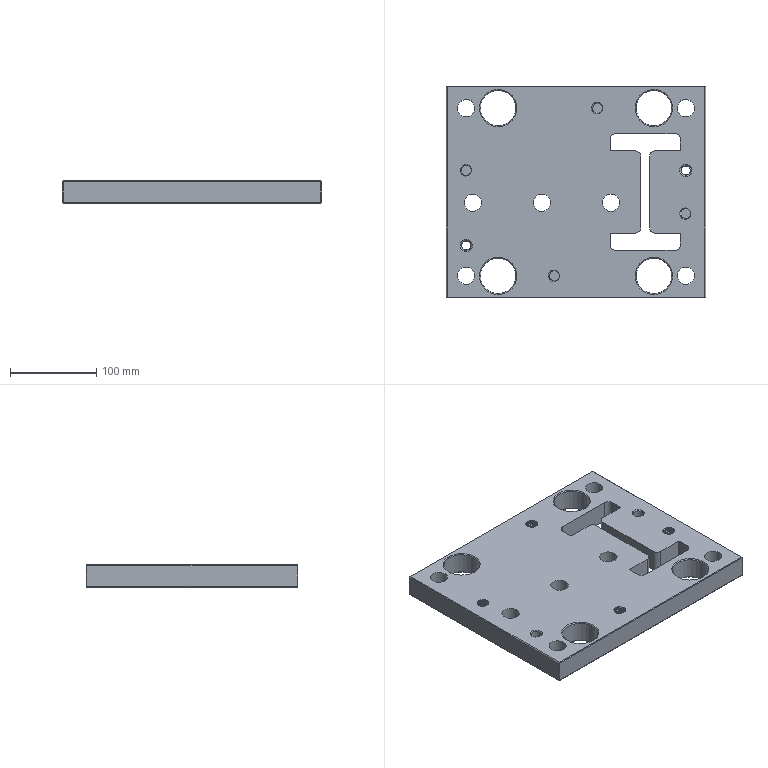Component | NX | PUNCH_HOLDER | 1 solid | 107 faces | volume 1589872 mm3 | plane 48 | cylinder 35 | spline 12 | cone 12 | commonest cylinder face diameters 12 x7 20.015 x7 41 x4 14 x4 11.985 x4 12.015 x3 1.015 x3 10.2 x2